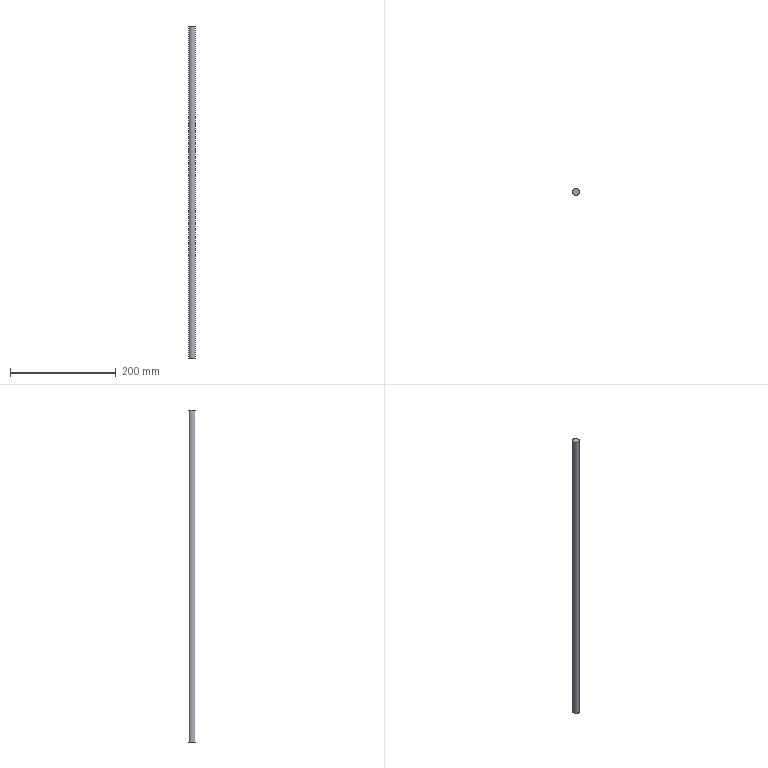Component | NX | SHAFT | 1 solid | 3 faces | box 12.7 x 12.7 x 627 mm | volume 79426 mm3 | plane 2 | cylinder 1 | commonest cylinder face diameters 12.7 x1
STEP:
#1=CARTESIAN_POINT('',(0.,0.,0.));
#2=DIRECTION('',(0.,0.,1.));
#3=DIRECTION('',(1.,0.,0.));
#4=AXIS2_PLACEMENT_3D('',#1,#2,#3);
#5=CARTESIAN_POINT('',(6.35,0.,627.));
#6=VERTEX_POINT('',#5);
#7=CARTESIAN_POINT('',(0.,0.,627.));
#8=DIRECTION('',(0.,0.,-1.));
#9=DIRECTION('',(1.,0.,0.));
#10=AXIS2_PLACEMENT_3D('',#7,#8,#9);
#11=CIRCLE('',#10,6.35);
#12=CARTESIAN_POINT('',(0.,0.,627.));
#13=DIRECTION('',(0.,0.,1.));
#14=DIRECTION('',(1.,0.,0.));
#15=AXIS2_PLACEMENT_3D('',#12,#13,#14);
#16=PLANE('',#15);
#17=CARTESIAN_POINT('',(6.35,0.));
#18=CARTESIAN_POINT('',(6.35,-10.999));
#19=CARTESIAN_POINT('',(-3.175,-5.499));
#20=CARTESIAN_POINT('',(-12.7,-0.));
#21=CARTESIAN_POINT('',(-3.175,5.499));
#22=CARTESIAN_POINT('',(6.35,10.999));
#23=CARTESIAN_POINT('',(6.35,0.));
#24=(BOUNDED_CURVE()B_SPLINE_CURVE(2,(#17,#18,#19,#20,#21,#22,#23),.UNSPECIFIED.,.T.,.F.)B_SPLINE_CURVE_WITH_KNOTS((1,2,2,2,2,1),(-2.094,0.,2.094,4.189,6.283,8.378),.UNSPECIFIED.)CURVE()GEOMETRIC_REPRESENTATION_ITEM()RATIONAL_B_SPLINE_CURVE((1.,0.5,1.,0.5,1.,0.5,1.))REPRESENTATION_ITEM(''));
#25=(GEOMETRIC_REPRESENTATION_CONTEXT(2)PARAMETRIC_REPRESENTATION_CONTEXT()REPRESENTATION_CONTEXT('',''));
#26=DEFINITIONAL_REPRESENTATION('',(#24),#25);
#27=PCURVE('',#16,#26);
#28=CARTESIAN_POINT('',(0.,0.,0.));
#29=DIRECTION('',(0.,0.,1.));
#30=DIRECTION('',(1.,0.,0.));
#31=AXIS2_PLACEMENT_3D('',#28,#29,#30);
#32=CYLINDRICAL_SURFACE('',#31,6.35);
#33=CARTESIAN_POINT('',(6.283,627.));
#34=DIRECTION('',(-1.,0.));
#35=VECTOR('',#34,1.);
#36=LINE('',#33,#35);
#37=(GEOMETRIC_REPRESENTATION_CONTEXT(2)PARAMETRIC_REPRESENTATION_CONTEXT()REPRESENTATION_CONTEXT('',''));
#38=DEFINITIONAL_REPRESENTATION('',(#36),#37);
#39=PCURVE('',#32,#38);
#40=SURFACE_CURVE('',#11,(#27,#39),.PCURVE_S1.);
#41=EDGE_CURVE('',#6,#6,#40,.T.);
#42=ORIENTED_EDGE('',*,*,#41,.F.);
#43=EDGE_LOOP('',(#42));
#44=FACE_BOUND('',#43,.T.);
#45=ADVANCED_FACE('',(#44),#16,.T.);
#46=CARTESIAN_POINT('',(6.35,0.,0.));
#47=VERTEX_POINT('',#46);
#48=CARTESIAN_POINT('',(0.,0.,0.));
#49=DIRECTION('',(0.,0.,1.));
#50=DIRECTION('',(1.,0.,0.));
#51=AXIS2_PLACEMENT_3D('',#48,#49,#50);
#52=CIRCLE('',#51,6.35);
#53=CARTESIAN_POINT('',(0.,0.,0.));
#54=DIRECTION('',(0.,0.,-1.));
#55=DIRECTION('',(-1.,0.,0.));
#56=AXIS2_PLACEMENT_3D('',#53,#54,#55);
#57=PLANE('',#56);
#58=CARTESIAN_POINT('',(-6.35,0.));
#59=CARTESIAN_POINT('',(-6.35,10.999));
#60=CARTESIAN_POINT('',(3.175,5.499));
#61=CARTESIAN_POINT('',(12.7,0.));
#62=CARTESIAN_POINT('',(3.175,-5.499));
#63=CARTESIAN_POINT('',(-6.35,-10.999));
#64=CARTESIAN_POINT('',(-6.35,0.));
#65=(BOUNDED_CURVE()B_SPLINE_CURVE(2,(#58,#59,#60,#61,#62,#63,#64),.UNSPECIFIED.,.T.,.F.)B_SPLINE_CURVE_WITH_KNOTS((1,2,2,2,2,1),(-2.094,0.,2.094,4.189,6.283,8.378),.UNSPECIFIED.)CURVE()GEOMETRIC_REPRESENTATION_ITEM()RATIONAL_B_SPLINE_CURVE((1.,0.5,1.,0.5,1.,0.5,1.))REPRESENTATION_ITEM(''));
#66=(GEOMETRIC_REPRESENTATION_CONTEXT(2)PARAMETRIC_REPRESENTATION_CONTEXT()REPRESENTATION_CONTEXT('',''));
#67=DEFINITIONAL_REPRESENTATION('',(#65),#66);
#68=PCURVE('',#57,#67);
#69=CARTESIAN_POINT('',(0.,0.));
#70=DIRECTION('',(1.,0.));
#71=VECTOR('',#70,1.);
#72=LINE('',#69,#71);
#73=(GEOMETRIC_REPRESENTATION_CONTEXT(2)PARAMETRIC_REPRESENTATION_CONTEXT()REPRESENTATION_CONTEXT('',''));
#74=DEFINITIONAL_REPRESENTATION('',(#72),#73);
#75=PCURVE('',#32,#74);
#76=SURFACE_CURVE('',#52,(#68,#75),.PCURVE_S1.);
#77=EDGE_CURVE('',#47,#47,#76,.T.);
#78=ORIENTED_EDGE('',*,*,#77,.F.);
#79=EDGE_LOOP('',(#78));
#80=FACE_BOUND('',#79,.T.);
#81=ADVANCED_FACE('',(#80),#57,.T.);
#82=ORIENTED_EDGE('',*,*,#41,.T.);
#83=CARTESIAN_POINT('',(6.35,-0.,0.));
#84=CARTESIAN_POINT('',(6.35,-0.,627.));
#85=B_SPLINE_CURVE_WITH_KNOTS('',1,(#83,#84),.UNSPECIFIED.,.F.,.F.,(2,2),(0.,627.),.PIECEWISE_BEZIER_KNOTS.);
#86=CARTESIAN_POINT('',(0.,0.));
#87=DIRECTION('',(0.,1.));
#88=VECTOR('',#87,1.);
#89=LINE('',#86,#88);
#90=(GEOMETRIC_REPRESENTATION_CONTEXT(2)PARAMETRIC_REPRESENTATION_CONTEXT()REPRESENTATION_CONTEXT('',''));
#91=DEFINITIONAL_REPRESENTATION('',(#89),#90);
#92=PCURVE('',#32,#91);
#93=CARTESIAN_POINT('',(6.283,0.));
#94=DIRECTION('',(0.,1.));
#95=VECTOR('',#94,1.);
#96=LINE('',#93,#95);
#97=(GEOMETRIC_REPRESENTATION_CONTEXT(2)PARAMETRIC_REPRESENTATION_CONTEXT()REPRESENTATION_CONTEXT('',''));
#98=DEFINITIONAL_REPRESENTATION('',(#96),#97);
#99=PCURVE('',#32,#98);
#100=SEAM_CURVE('',#85,(#92,#99),.PCURVE_S1.);
#101=EDGE_CURVE('',#47,#6,#100,.T.);
#102=ORIENTED_EDGE('',*,*,#101,.F.);
#103=ORIENTED_EDGE('',*,*,#77,.T.);
#104=ORIENTED_EDGE('',*,*,#101,.T.);
#105=EDGE_LOOP('',(#82,#102,#103,#104));
#106=FACE_BOUND('',#105,.T.);
#107=ADVANCED_FACE('',(#106),#32,.T.);
#108=CLOSED_SHELL('',(#45,#81,#107));
#109=MANIFOLD_SOLID_BREP('',#108);
#110=(LENGTH_UNIT()NAMED_UNIT(*)SI_UNIT(.MILLI.,.METRE.));
#111=UNCERTAINTY_MEASURE_WITH_UNIT(LENGTH_MEASURE(0.00001),#110,'','');
#112=(NAMED_UNIT(*)PLANE_ANGLE_UNIT()SI_UNIT($,.RADIAN.));
#113=(NAMED_UNIT(*)SI_UNIT($,.STERADIAN.)SOLID_ANGLE_UNIT());
#114=(GEOMETRIC_REPRESENTATION_CONTEXT(3)GLOBAL_UNCERTAINTY_ASSIGNED_CONTEXT((#111))GLOBAL_UNIT_ASSIGNED_CONTEXT((#110,#112,#113))REPRESENTATION_CONTEXT('',''));
#115=ADVANCED_BREP_SHAPE_REPRESENTATION('',(#4,#109),#114);